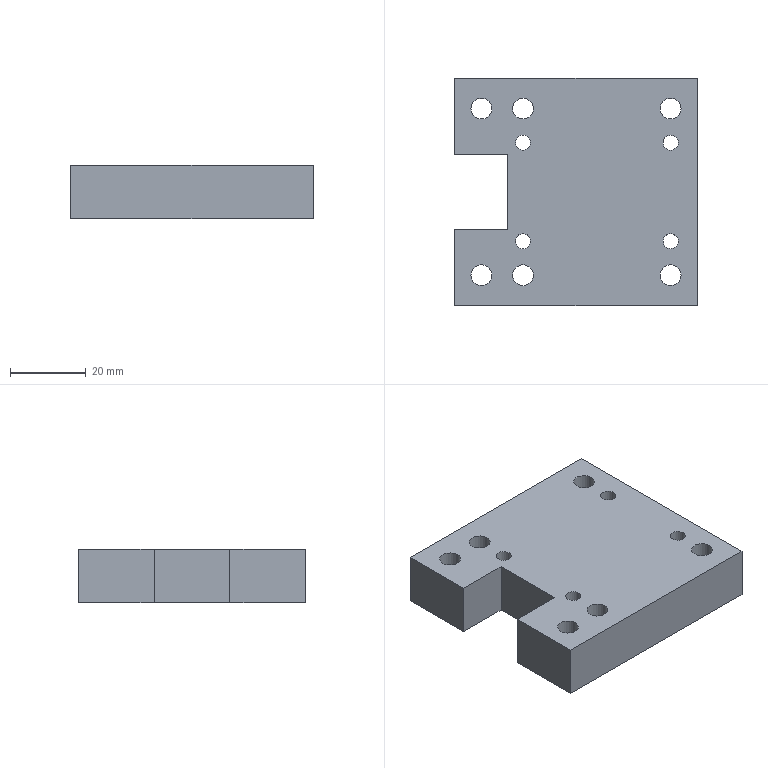Component | NX | 1_BASE_PLATE | 1 solid | 32 faces | volume 45444 mm3 | plane 16 | cylinder 16 | commonest cylinder face diameters 5.5 x6 9.5 x6 4 x4